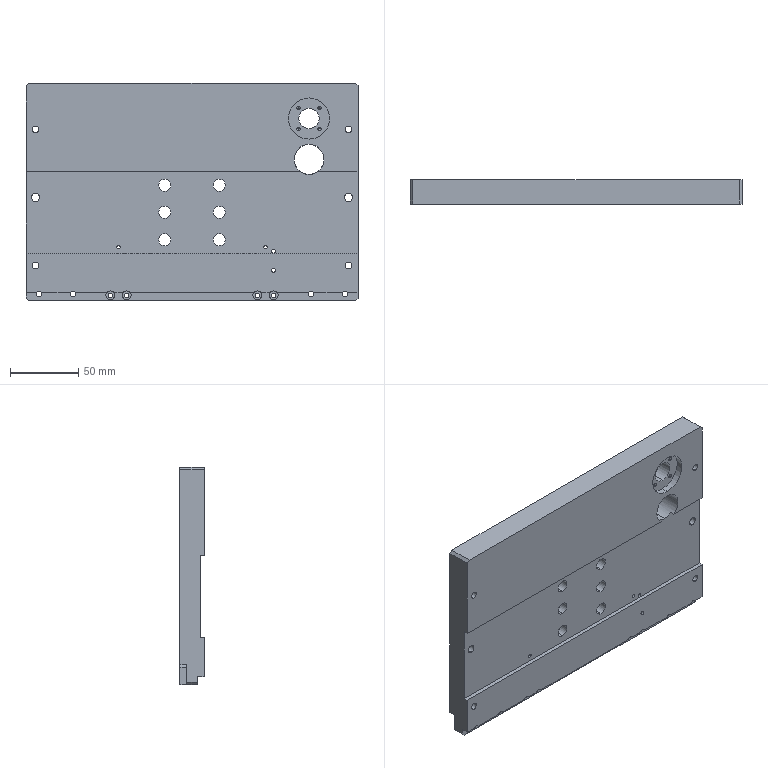Component | SolidWorks | SAWH02-03101A0MountingPlate1-2 | 1 solid | 156 faces | box 244 x 18 x 160 mm | volume 597572 mm3 | cylinder 94 | plane 50 | cone 12 | commonest cylinder face diameters 2.5 x16 15 x14 9 x12 3.4 x8 6.5 x8 4.2 x8 6 x8 5 x8 | material 6061
build123d program:
from build123d import *

# Parameters (mm, degrees)
SKETCH1_W                                       = 244
SKETCH1_H                                       = 160
BOSS_EXTRUDE1_DEPTH                             = 18
CHAMFER1_SIZE                                   = 2
CUT_EXTRUDE5_DEPTH                              = 8
M3_TAPPED_HOLE2_D                               = 2.5
M3_TAPPED_HOLE2_DEPTH                           = 7.5
M3_TAPPED_HOLE2_TIP                             = 0.7511
SKETCH83_R                                      = 1.5
CUT_EXTRUDE3_DEPTH                              = 30
M8_HEX_SOCKET_HEAD_CAP_SCREW_CBORE1_D           = 9
M8_HEX_SOCKET_HEAD_CAP_SCREW_CBORE1_CBORE_D     = 15
M8_HEX_SOCKET_HEAD_CAP_SCREW_CBORE1_CBORE_DEPTH = 8.6
M6_TAPPED_HOLE2_D                               = 5
F_6_0_6_DIAMETER_HOLE1_D                        = 6
F_6_0_6_DIAMETER_HOLE1_DEPTH                    = 15
F_6_0_6_DIAMETER_HOLE1_TIP                      = 1.803
SKETCH118_W                                     = 44
SKETCH118_H                                     = 15
CUT_EXTRUDE8_DEPTH                              = 5
SKETCH134_R                                     = 2
CUT_EXTRUDE14_DEPTH                             = 5
M5_TAPPED_HOLE3_D                               = 4.2
SKETCH122_R                                     = 7.5
CUT_EXTRUDE10_DEPTH                             = 203.01
SKETCH121_R                                     = 11
CUT_EXTRUDE9_DEPTH                              = 203.01
SKETCH123_W                                     = 6
SKETCH123_H                                     = 5
CUT_EXTRUDE11_DEPTH                             = 293.335
M3_HEX_SOCKET_HEAD_CAP_SCREW_CBORE1_D           = 3.4
M3_HEX_SOCKET_HEAD_CAP_SCREW_CBORE1_CBORE_D     = 6.5
M3_HEX_SOCKET_HEAD_CAP_SCREW_CBORE1_CBORE_DEPTH = 8
SKETCH129_R                                     = 15.1
CUT_EXTRUDE12_DEPTH                             = 5
M3_TAPPED_HOLE3_D                               = 2.5
M3_TAPPED_HOLE3_DEPTH                           = 7.5
M3_TAPPED_HOLE3_TIP                             = 0.7511
SKETCH133_W                                     = 244
SKETCH133_H                                     = 60
CUT_EXTRUDE13_DEPTH                             = 3


with BuildPart() as part:
    # Sketch1 → Boss-Extrude1 (new body)
    with BuildSketch(Plane(origin=(0, 0, 0), x_dir=(1, 0, 0), z_dir=(0, 1, 0))):
        with Locations((0, 80)):
            Rectangle(SKETCH1_W, SKETCH1_H)
    extrude(amount=BOSS_EXTRUDE1_DEPTH)

    # Chamfer1
    chamfer1_edges = [part.edges().sort_by_distance(p)[0] for p in [
        (-122, 9, -160),
        (122, 9, -160),
        (122, 9, 0),
        (-122, 9, 0),
    ]]
    chamfer(chamfer1_edges, length=CHAMFER1_SIZE)

    # Sketch104 → Cut-Extrude5 (cut)
    with BuildSketch(Plane(origin=(0, 18, 0), x_dir=(1, 0, 0), z_dir=(0, 1, 0))):
        with BuildLine():
            Line((-66, 160), (-42, 160))
            Line((-42, 160), (-42, 113))
            ThreePointArc((-42, 113), (-42.879, 110.879), (-45, 110))
            Line((-45, 110), (-63, 110))
            ThreePointArc((-63, 110), (-65.121, 110.879), (-66, 113))
            Line((-66, 113), (-66, 160))
        make_face()
        with BuildLine():
            Line((45, 110), (63, 110))
            ThreePointArc((63, 110), (65.121, 110.879), (66, 113))
            Line((66, 113), (66, 160))
            Line((66, 160), (42, 160))
            Line((42, 160), (42, 113))
            ThreePointArc((42, 113), (42.879, 110.879), (45, 110))
        make_face()
    extrude(amount=-CUT_EXTRUDE5_DEPTH, mode=Mode.SUBTRACT)

    # M3 Tapped Hole2
    with Locations(Plane(origin=(0, 10, 0), x_dir=(1, 0, 0), z_dir=(0, 1, 0))):
        with Locations((54, 120.5), (54, 140.5), (-54, 140.5), (-54, 120.5)):
            Hole(M3_TAPPED_HOLE2_D / 2, depth=M3_TAPPED_HOLE2_DEPTH)
            with Locations((0, 0, -(M3_TAPPED_HOLE2_DEPTH + M3_TAPPED_HOLE2_TIP / 2))):  # 118° drill point
                Cone(0, M3_TAPPED_HOLE2_D / 2, M3_TAPPED_HOLE2_TIP, mode=Mode.SUBTRACT)

    # Sketch83 → Cut-Extrude3 (cut)
    with BuildSketch(Plane(origin=(0, 10, 0), x_dir=(1, 0, 0), z_dir=(0, 1, 0))):
        with Locations(Location((60, 137.5, 0), (0, 0, 270))):
            Circle(SKETCH83_R)
        with Locations(Location((60, 123.5, 0), (0, 0, 90))):
            Circle(SKETCH83_R)
    extrude(amount=-CUT_EXTRUDE3_DEPTH, mode=Mode.SUBTRACT)

    # M8 Hex Socket Head Cap Screw CBORE1 (through all)
    with Locations(Plane(origin=(0, 18, 0), x_dir=(1, 0, 0), z_dir=(0, 1, 0))):
        with Locations((20, 75), (-20, 75), (-20, 115), (20, 115), (-20, 95), (20, 95)):
            CounterBoreHole(M8_HEX_SOCKET_HEAD_CAP_SCREW_CBORE1_D / 2, M8_HEX_SOCKET_HEAD_CAP_SCREW_CBORE1_CBORE_D / 2, M8_HEX_SOCKET_HEAD_CAP_SCREW_CBORE1_CBORE_DEPTH)

    # M6 Tapped Hole2 (through all)
    with Locations(Plane(origin=(0, 18, 0), x_dir=(1, 0, 0), z_dir=(0, 1, 0))):
        with Locations((-115, 134), (-115, 34), (115, 34), (115, 134)):
            Hole(M6_TAPPED_HOLE2_D / 2)

    # 6.0 _6_ Diameter Hole1
    with Locations(Plane(origin=(0, 18, 0), x_dir=(1, 0, 0), z_dir=(0, 1, 0))):
        with Locations((-115, 84), (115, 84)):
            Hole(F_6_0_6_DIAMETER_HOLE1_D / 2, depth=F_6_0_6_DIAMETER_HOLE1_DEPTH)
            with Locations((0, 0, -(F_6_0_6_DIAMETER_HOLE1_DEPTH + F_6_0_6_DIAMETER_HOLE1_TIP / 2))):  # 118° drill point
                Cone(0, F_6_0_6_DIAMETER_HOLE1_D / 2, F_6_0_6_DIAMETER_HOLE1_TIP, mode=Mode.SUBTRACT)

    # Sketch118 → Cut-Extrude8 (cut)
    with BuildSketch(Plane(origin=(0, 18, 0), x_dir=(1, 0, 0), z_dir=(0, 1, 0))):
        with Locations((100, 152.5)):
            Rectangle(SKETCH118_W, SKETCH118_H)
        with Locations((-100, 152.5)):
            Rectangle(SKETCH118_W, SKETCH118_H)
    extrude(amount=-CUT_EXTRUDE8_DEPTH, mode=Mode.SUBTRACT)

    # Sketch134 → Cut-Extrude14 (cut)
    with BuildSketch(Plane(origin=(0, 18, 0), x_dir=(1, 0, 0), z_dir=(0, 1, 0))):
        with Locations((-78, 145)):
            Circle(SKETCH134_R)
        with Locations((78, 145)):
            Circle(SKETCH134_R)
    extrude(amount=-CUT_EXTRUDE14_DEPTH, mode=Mode.SUBTRACT)

    # M5 Tapped Hole3 (through all)
    with Locations(Plane(origin=(0, 13, 0), x_dir=(1, 0, 0), z_dir=(0, 1, 0))):
        with Locations((-112.5, 155), (-87.5, 155), (87.5, 155), (112.5, 155)):
            Hole(M5_TAPPED_HOLE3_D / 2)

    # Sketch122 → Cut-Extrude10 (cut, through all)
    with BuildSketch(Plane.XZ):
        with Locations(Location((86, -26, 0), (0, 0, 270))):
            Circle(SKETCH122_R)
    extrude(amount=-CUT_EXTRUDE10_DEPTH, mode=Mode.SUBTRACT)

    # Sketch121 → Cut-Extrude9 (cut, through all)
    with BuildSketch(Plane(origin=(0, 18, 0), x_dir=(1, 0, 0), z_dir=(0, 1, 0))):
        with Locations(Location((86, 56, 0), (0, 0, 270))):
            Circle(SKETCH121_R)
    extrude(amount=-CUT_EXTRUDE9_DEPTH, mode=Mode.SUBTRACT)

    # Sketch123 → Cut-Extrude11 (cut, through all)
    with BuildSketch(Plane.ZY.offset(122)):
        with Locations((-157, 2.5)):
            Rectangle(SKETCH123_W, SKETCH123_H)
    extrude(amount=-CUT_EXTRUDE11_DEPTH, mode=Mode.SUBTRACT)

    # M3 Hex Socket Head Cap Screw CBORE1 (through all)
    with Locations(Plane(origin=(0, 0, 0), x_dir=(-1, 0, 0), z_dir=(0, -1, 0))):
        with Locations((-60, 156), (-48, 156), (48, 156), (60, 156)):
            CounterBoreHole(M3_HEX_SOCKET_HEAD_CAP_SCREW_CBORE1_D / 2, M3_HEX_SOCKET_HEAD_CAP_SCREW_CBORE1_CBORE_D / 2, M3_HEX_SOCKET_HEAD_CAP_SCREW_CBORE1_CBORE_DEPTH)

    # Sketch129 → Cut-Extrude12 (cut)
    with BuildSketch(Plane(origin=(0, 0, 0), x_dir=(1, 0, 0), z_dir=(0, 1, 0))):
        with Locations(Location((86, 26, 0), (0, 0, 270))):
            Circle(SKETCH129_R)
    extrude(amount=CUT_EXTRUDE12_DEPTH, mode=Mode.SUBTRACT)

    # M3 Tapped Hole3
    with Locations(Plane(origin=(0, 5, 0), x_dir=(-1, 0, 0), z_dir=(0, -1, 0))):
        with Locations((-78.222, 18.222), (-93.778, 18.222), (-93.778, 33.778), (-78.222, 33.778)):
            Hole(M3_TAPPED_HOLE3_D / 2, depth=M3_TAPPED_HOLE3_DEPTH)
            with Locations((0, 0, -(M3_TAPPED_HOLE3_DEPTH + M3_TAPPED_HOLE3_TIP / 2))):  # 118° drill point
                Cone(0, M3_TAPPED_HOLE3_D / 2, M3_TAPPED_HOLE3_TIP, mode=Mode.SUBTRACT)

    # Sketch133 → Cut-Extrude13 (cut)
    with BuildSketch(Plane.XZ):
        with Locations((0, -95)):
            Rectangle(SKETCH133_W, SKETCH133_H)
    extrude(amount=-CUT_EXTRUDE13_DEPTH, mode=Mode.SUBTRACT)


solid = part.part

# Placed as in the assembly
solid = solid.moved(Location((27.51, -30.388, 21.208), (0, 0, 0)))